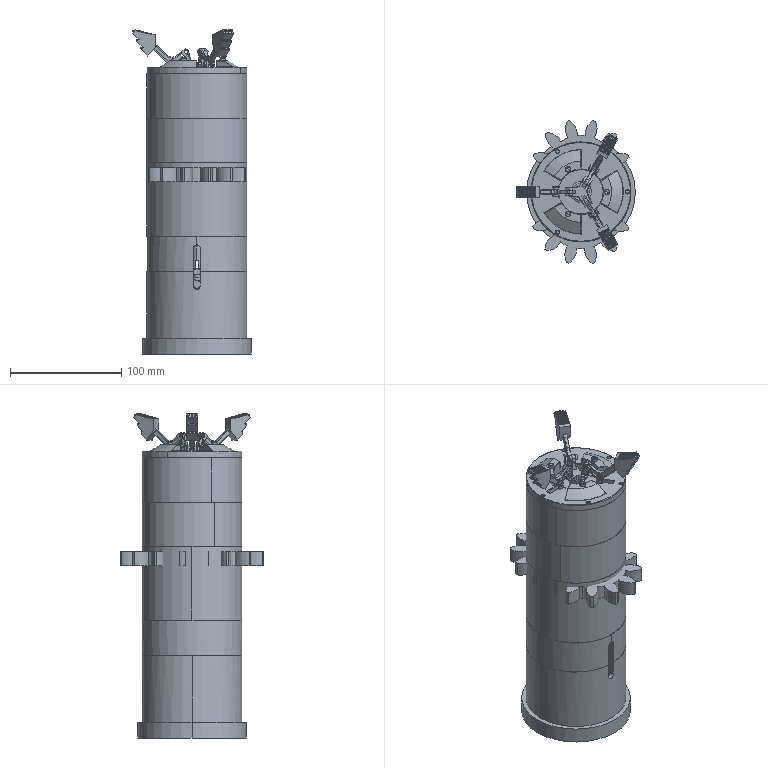Assembly | SolidWorks | mm | 29 component files | 29 solids | 1673 faces | box 106.87 x 128.59 x 291.77 mm | volume 704816 mm3 | cylinder 802 | plane 633 | torus 98 | cone 78 | spline 42 | sphere 20 | commonest cylinder face diameters 1 x109 30.48 x84 3 x76 5 x73 1.5 x54 4 x43 60.322 x39 8 x38
Bill of materials:
Cam2 | 1 |  | Thin-walled cylindrical cup with a flat closed floor and a small central through-hole; the open rim is cut on a slant, so the wall height varies around the circumference.
g | 1 |  | T-shaped body: a long vertical round shaft that meets a horizontal cylindrical crossbar with chamfered ends. The shaft has an annular collar partway up, a section split by longitudinal grooves or slots near the top, and a top head with several radial tabs, each with a through-hole.
g1 | 1 |  | Open-top cylindrical cup with a wider base flange, a small stepped lip at the top, and two opposed vertical slots with rounded ends cut down from the rim. The floor has a central round hole surrounded by four small holes in a square pattern.
g11 | 1 |  | Open-top cylindrical cup with a stepped, slightly narrower lip at the top rim and plain outer wall. The floor has a large central hole and four small holes in a square pattern.
g2 | 1 |  | Short, wide cylindrical cup with a reduced-diameter step at the top rim and a flat floor with one small central through-hole. A shallow ring or counterbore surrounds the hole.
GMotor | 2 |  | Boxy body with a square cross-section between a large square top plate and a smaller square bottom flange. The top plate has four small corner holes, a raised square pad, concentric annular recesses or bosses, and a short central cylindrical shaft stub. The vertical corners have rounded grooves, the bottom flange has corner holes, and a small cylindrical nub sticks out low on one side.
GMotorAxis | 2 |  | Solid stepped cylindrical pin: a larger-diameter lower section with a chamfered bottom edge and a smaller-diameter upper section. A small flat or notch appears on one side of the upper section.
GMotorCover | 1 |  | Shallow round tray with a thin vertical wall, a thin outward-flaring rim flange at the top, and two opposed rounded-end vertical slots cut from the rim. The floor has a central rounded-square opening, four small holes around it, and a tiny center hole.
GMotorCover2 | 1 |  | Shallow round tray like the slotted variant but with no wall slots. It has a thin flared top rim, a central rounded-square floor opening, four small holes in a square pattern, and two additional larger round holes on opposite sides of the opening.
GRingCam | 2 |  | Thin-walled cylindrical cup with a flat floor and a central through-hole. The open rim is cut on a steep slant, so the wall runs from low on one side to tall on the other.
GuideCover | 1 |  | Short cylindrical puck or cap with a raised, slightly smaller top face that has a chamfered edge. At the center is a counterbored through-hole, and one vertical slot with a rounded end is cut into the side wall from the bottom edge.
GuideRod1 | 1 |  | Stepped cylindrical shaft: a smaller-diameter upper pin with a chamfered end above a longer main body. The lower end is split into a clevis-like fork by a slot, and a transverse through-hole crosses the fork near its rounded or chamfered end.
hex nuts, style 1-grades ab gb | 2 |  | Hexagonal prism with a central cylindrical through-bore and chamfered corners at both ends; looks like a hex nut.
Jaw2 | 3 |  | Lever-like part: a rectangular block with stepped sides, with parallel grooves on one face and three small round pins sticking out of one end. A slender arm comes off the block and bends toward an end with holed lugs or eyes, which form a fork in one view.
JawCover | 1 |  | Flat round flange plate with a large central opening and six small through-holes spaced evenly near the rim. On top are three raised sector pads with sloped outer faces, each carrying a short round boss. Between the pads are three radial through-slots, each with a pair of small holed lugs beside it.
JawOne | 3 |  | Flat link plate with rounded ends (obround outline) and one round through-hole at each end. A long shallow recess or slot runs between the holes on one face.
SpringCover | 1 |  | Shallow round cup with a thick wall and open top. A short round hub boss with a central through-hole sits at the center of the floor.
spur gear_gb | 3 |  | Flat spur-gear-like disk with 12 rounded, lobe-shaped teeth and a central round bore.
WasherM6 | 1 |  | Thin flat annular ring (plain washer-like disc) with a concentric through-bore and a small chamfer on the outer edge of one face.
Mates:
1. concentric | g1-1 face at (-15.928, -1.7, 30) dir (0, 0, -1) r 45 | GMotor-1 face at (-15.928, -1.7, 16) dir (0, 0, -1) r 2.5
2. coincident | g1-1 face at (-60.928, -1.7, -22) dir (0, 0, 1) | GMotor-1 face at (-15.928, -1.7, -22) dir (0, 0, -1)
3. concentric | g1-1 face at (-27.928, 10.3, -15) dir (0, 0, -1) r 2 | GMotor-1 face at (-27.928, 10.3, -22) dir (0, 0, -1) r 0.889
4. concentric | g1-1 face at (-15.928, -1.7, 30) dir (0, 0, -1) r 45 | GMotorCover-2 face at (-15.928, -1.7, 13) dir (0, 0, -1) r 40.5
5. parallel | GMotor-1 face at (1.572, -19.2, 11) dir (0, -1, 0) | GMotorCover-2 face at (-25.528, -15.3, 11) dir (0, 1, 0)
6. coincident | GMotor-1 face at (-15.928, -1.7, 11) dir (0, 0, 1) | GMotorCover-2 face at (-15.928, -1.7, 11) dir (0, 0, -1)
7. concentric | g1-1 face at (-15.928, -1.7, 30) dir (0, 0, -1) r 45 | GMotorAxis-1 face at (-15.928, -1.7, 27) dir (0, 0, -1) r 3
8. coincident | GMotor-1 face at (-15.928, -1.7, 11) dir (0, 0, 1) | GMotorAxis-1 face at (-15.928, -1.7, 11) dir (0, 0, -1)
9. concentric | GMotorCover-2 face at (-15.928, -1.7, 36) dir (0, 0, -1) r 39 | WasherM6-1 face at (-15.928, -1.7, 15.055) dir (0, 0, 1) r 6
10. coincident | WasherM6-1 face at (-15.928, -1.7, 16.655) dir (0, 0, 1) | hex nuts, style 1-grades ab gb-2 face at (-19.199, -10.339, 16.655) dir (0, 0, -1)
11. concentric | WasherM6-1 face at (-15.928, -1.7, 15.055) dir (0, 0, 1) r 6 | hex nuts, style 1-grades ab gb-2 face at (-15.928, -1.7, 16.655) dir (0, 0, 1) r 4.5
12. concentric | GMotorAxis-1 face at (-15.928, -1.7, 27) dir (0, 0, -1) r 3 | Cam2-1 face at (-15.928, -1.7, 35.055) dir (0, 0, -1) r 21
13. coincident | WasherM6-1 face at (-15.928, -1.7, 15.055) dir (0, 0, -1) | Cam2-1 face at (-15.928, -1.7, 15.055) dir (0, 0, 1)
14. concentric | Cam2-1 face at (-15.928, -1.7, 35.055) dir (0, 0, -1) r 19 | GuideCover-1 face at (-15.928, -1.7, 66) dir (0, 0, -1) r 45
15. coincident | g1-1 face at (-15.928, -1.7, 30) dir (0, 0, 1) | GuideCover-1 face at (-15.928, -1.7, 30) dir (0, 0, -1)
16. concentric | g1-1 face at (-15.928, -1.7, 30) dir (0, 0, -1) r 45 | GuideRod1-1 face at (-15.928, -1.7, 32) dir (0, 0, 1) r 4
17. coincident | GuideCover-1 face at (-15.928, -1.7, 62) dir (0, 0, -1) | GuideRod1-1 face at (-15.928, -1.7, 62) dir (0, 0, 1)
18. parallel | GMotor-1 face at (-30.928, -16.7, -22) dir (-1, 0, 0) | GuideRod1-1 face at (-17.428, -14.7, 24) dir (1, 0, 0)
19. parallel | g1-1 face at (-13.137, -131.7, 14) dir (-1, 0, 0) | GuideCover-1 face at (-12.928, 88.3, 6) dir (-1, 0, 0)
20. concentric | GuideRod1-1 face at (-15.928, -1.7, 70) dir (0, 0, -1) r 2.458 | hex nuts, style 1-grades ab gb-3 face at (-15.928, -1.7, 64) dir (0, 0, 1) r 4.5
21. coincident | GuideCover-1 face at (-15.928, -1.7, 64) dir (0, 0, 1) | hex nuts, style 1-grades ab gb-3 face at (-10.637, 5.872, 64) dir (0, 0, -1)
22. concentric | g1-1 face at (-15.928, -1.7, 30) dir (0, 0, -1) r 45 | g11-1 face at (-15.928, -1.7, 128) dir (0, 0, -1) r 45
23. coincident | GuideCover-1 face at (-60.928, -1.7, 62) dir (0, 0, 1) | g11-1 face at (-15.928, -1.7, 62) dir (0, 0, -1)
24. lock | GuideCover-1 reference at (0, 0, 0) dir (1, 0, 0) | g11-1 reference at (0, 0, 0) dir (1, 0, 0)
25. concentric | g11-1 face at (-15.928, -1.7, 128) dir (0, 0, -1) r 45 | GMotor-2 face at (-15.928, -1.7, 114) dir (0, 0, -1) r 2.5
26. concentric | g11-1 face at (-27.928, 10.3, 83) dir (0, 0, -1) r 2 | GMotor-2 face at (-27.928, 10.3, 76) dir (0, 0, -1) r 0.889
27. coincident | g11-1 face at (-60.928, -1.7, 76) dir (0, 0, 1) | GMotor-2 face at (-15.928, -1.7, 76) dir (0, 0, -1)
28. concentric | g11-1 face at (-15.928, -1.7, 128) dir (0, 0, -1) r 45 | GMotorCover2-1 face at (-15.928, -1.7, 111) dir (0, 0, -1) r 40.5
29. parallel | GMotor-2 face at (1.572, 15.8, 109) dir (1, 0, 0) | GMotorCover2-1 face at (-2.328, 7.9, 109) dir (-1, 0, 0)
30. coincident | g11-1 edge at (-15.928, -1.7, 134) dir (0, 0, -1) r 43 | GMotorCover2-1 face at (-15.928, -1.7, 134) dir (0, 0, -1)
31. concentric | g11-1 face at (-15.928, -1.7, 128) dir (0, 0, -1) r 45 | spur gear_gb-7 face at (-15.928, -1.7, 98.3) dir (0, 0, 1) r 9.525
32. coincident | GMotorCover2-1 face at (-15.928, -1.7, 111) dir (0, 0, 1) | spur gear_gb-7 face at (-15.928, -1.7, 111) dir (0, 0, -1)
33. concentric | GMotorCover2-1 face at (-15.928, 19.3, 119) dir (0, 0, -1) r 3 | spur gear_gb-5 face at (-15.928, 19.3, 136.4) dir (0, 0, -1) r 9.525
34. coincident | GMotorCover2-1 face at (-15.928, -1.7, 111) dir (0, 0, 1) | spur gear_gb-5 face at (-15.928, 19.3, 111) dir (0, 0, -1)
35. concentric | GMotorCover2-1 face at (-15.928, -22.7, 119) dir (0, 0, -1) r 3 | spur gear_gb-6 face at (-15.928, -22.7, 98.3) dir (0, 0, 1) r 9.525
36. coincident | GMotorCover2-1 face at (-15.928, -1.7, 111) dir (0, 0, 1) | spur gear_gb-6 face at (-15.928, -22.7, 111) dir (0, 0, -1)
37. concentric | g11-1 face at (-15.928, -1.7, 128) dir (0, 0, -1) r 45 | GMotorAxis-2 face at (-15.928, -1.7, 125.3) dir (0, 0, -1) r 3
38. coincident | GMotor-2 face at (-6.428, -11.202, 109.3) dir (0, 0, 1) | GMotorAxis-2 face at (-15.928, -1.7, 109.3) dir (0, 0, -1)
39. coincident | spur gear_gb-7 face at (-19.811, -3.086, 67) dir (-0.09773, 0.9952, 0) | GMotorAxis-2 face at (-17.821, -2.891, 111.3) dir (-0.09773, 0.9952, 0)
40. gear | spur gear_gb-6 face at (-15.928, -22.7, 111) dir (0, 0, 1) r 30.161 | spur gear_gb-7 face at (-15.928, -1.7, 111) dir (0, 0, 1) r 30.161
41. gear | spur gear_gb-7 face at (-15.928, -1.7, 111) dir (0, 0, 1) r 30.161 | spur gear_gb-5 face at (-15.928, 19.3, 123.7) dir (0, 0, -1) r 30.161
42. concentric | spur gear_gb-5 face at (-15.928, 19.3, 136.4) dir (0, 0, -1) r 9.525 | GRingCam-10 face at (-15.928, 19.3, 133) dir (0, 0, -1) r 18
43. coincident | spur gear_gb-5 face at (-15.928, 19.3, 123.7) dir (0, 0, 1) | GRingCam-10 face at (-15.928, 19.3, 117) dir (0, 0, -1)
44. lock | spur gear_gb-5 reference at (0, 0, 0) dir (1, 0, 0) | GRingCam-10 reference at (0, 0, 0) dir (1, 0, 0)
45. concentric | spur gear_gb-6 face at (-15.928, -22.7, 98.3) dir (0, 0, 1) r 9.525 | GRingCam-8 face at (-15.928, -22.7, 139.7) dir (0, 0, -1) r 18
46. coincident | spur gear_gb-6 face at (-15.928, -22.7, 123.7) dir (0, 0, 1) | GRingCam-8 face at (-15.928, -22.7, 123.7) dir (0, 0, -1)
47. lock | spur gear_gb-6 reference at (0, 0, 0) dir (1, 0, 0) | GRingCam-8 reference at (0, 0, 0) dir (1, 0, 0)
48. concentric | g11-1 face at (-15.928, -1.7, 128) dir (0, 0, -1) r 45 | g-1 face at (-15.928, -1.7, 214.212) dir (0, 0, -1) r 6
49. parallel | GMotor-2 face at (-0.928, -16.7, 76) dir (0, -1, 0) | g-1 face at (-15.928, -21.7, 144.212) dir (0, -1, 0)
50. concentric | g1-1 face at (-15.928, -1.7, 30) dir (0, 0, -1) r 45 | g2-1 face at (-15.928, -1.7, 128) dir (0, 0, 1) r 45
51. coincident | g11-1 face at (-15.928, -1.7, 128) dir (0, 0, 1) | g2-1 face at (-15.928, -1.7, 128) dir (0, 0, -1)
52. concentric | g2-1 face at (-15.928, -1.7, 128) dir (0, 0, 1) r 45 | SpringCover-2 face at (-15.928, -1.7, 168) dir (0, 0, 1) r 45
53. coincident | g2-1 face at (-15.928, -1.7, 168) dir (0, 0, 1) | SpringCover-2 face at (-15.928, -1.7, 168) dir (0, 0, -1)
54. concentric | SpringCover-2 face at (-15.928, -1.7, 168) dir (0, 0, 1) r 45 | JawCover-1 face at (-15.928, -1.7, 214) dir (0, 0, -1) r 45
55. coincident | SpringCover-2 face at (-15.928, -1.7, 208) dir (0, 0, 1) | JawCover-1 face at (-15.928, -1.7, 208) dir (0, 0, -1)
56. parallel | g-1 face at (-12.365, 1.472, 190.212) dir (-0.866, 0.5, 0) | JawCover-1 face at (3.275, 27.561, 181) dir (-0.866, 0.5, 0)
57. concentric | g-1 face at (-23.175, 22.3, 216.212) dir (0, -1, 0) r 1.5 | JawOne-1 face at (-23.175, -3.2, 216.212) dir (0, 1, 0) r 1.5
58. coincident | g-1 face at (-20.457, -0.2002, 190.212) dir (0, -1, 0) | JawOne-1 face at (-23.175, -0.2002, 216.212) dir (0, 1, 0)
59. concentric | JawCover-1 face at (-38.428, -5.7, 218) dir (0, 1, 0) r 1.5 | Jaw2-1 face at (-38.428, 14.8, 218) dir (0, -1, 0) r 1.5
60. concentric | JawOne-1 face at (-25.864, -3.2, 227.907) dir (0, 1, 0) r 1.5 | Jaw2-1 face at (-25.864, 12.8, 227.907) dir (0, -1, 0) r 1.5
61. concentric | g-1 face at (8.48, -7.424, 216.212) dir (-0.866, 0.5, 0) r 1.5 | JawOne-3 face at (-13.604, 5.326, 216.212) dir (0.866, -0.5, 0) r 1.5
62. coincident | g-1 face at (-12.365, 1.472, 190.212) dir (-0.866, 0.5, 0) | JawOne-3 face at (-9.661, 6.155, 227.907) dir (0.866, -0.5, 0)
63. concentric | g-1 face at (-33.089, -19.976, 216.212) dir (0.866, 0.5, 0) r 1.5 | JawOne-4 face at (-11.006, -7.226, 216.212) dir (-0.866, -0.5, 0) r 1.5
64. coincident | g-1 face at (-12.365, -4.872, 190.212) dir (-0.866, -0.5, 0) | JawOne-4 face at (-11.006, -7.226, 216.212) dir (0.866, 0.5, 0)
65. concentric | JawOne-3 face at (-12.259, 7.655, 227.907) dir (0.866, -0.5, 0) r 1.5 | Jaw2-2 face at (1.597, -0.3455, 227.907) dir (-0.866, 0.5, 0) r 1.5
66. concentric | JawCover-1 face at (-8.142, 19.785, 218) dir (0.866, -0.5, 0) r 1.5 | Jaw2-2 face at (9.611, 9.535, 218) dir (-0.866, 0.5, 0) r 1.5
67. concentric | JawOne-4 face at (-9.661, -9.555, 227.907) dir (-0.866, -0.5, 0) r 1.5 | Jaw2-3 face at (-23.517, -17.555, 227.907) dir (0.866, 0.5, 0) r 1.5
68. concentric | JawCover-1 face at (-1.214, -19.186, 218) dir (-0.866, -0.5, 0) r 1.5 | Jaw2-3 face at (-18.967, -29.436, 218) dir (0.866, 0.5, 0) r 1.5
69. concentric | JawOne-3 face at (-12.259, 7.655, 227.907) dir (0.866, -0.5, 0) r 1.5 | Jaw2-2 face at (1.597, -0.3455, 227.907) dir (-0.866, 0.5, 0) r 1.5
70. distance | JawCover-1 face at (-17.083, -3.7, 181) dir (0, 1, 0) | Jaw2-1 face at (-38.428, -3.2, 218) dir (0, -1, 0)
71. distance | JawCover-1 face at (3.275, 27.561, 181) dir (-0.866, 0.5, 0) | Jaw2-2 face at (-3.379, 17.035, 218) dir (0.866, -0.5, 0)
72. distance | JawCover-1 face at (-13.619, -1.7, 181) dir (-0.866, -0.5, 0) | Jaw2-3 face at (-3.379, -20.436, 218) dir (0.866, 0.5, 0)